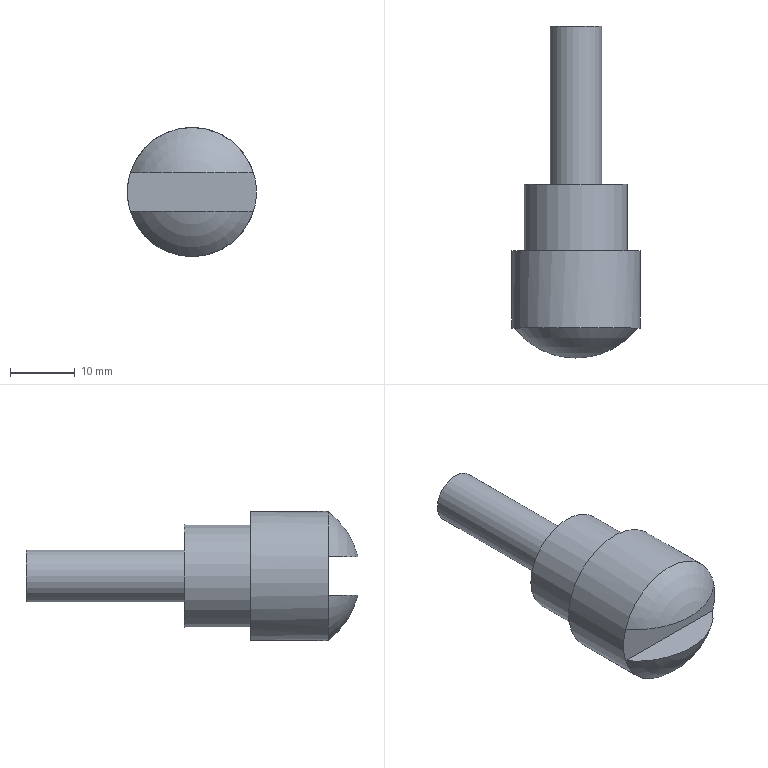Component | NX | 5_STUD | 1 solid | 11 faces | box 20 x 51.43 x 20 mm | volume 7520 mm3 | plane 6 | cylinder 3 | sphere 2 | commonest cylinder face diameters 20 x1 16 x1 8 x1
STEP:
#1=CARTESIAN_POINT('',(0.,0.,0.));
#2=DIRECTION('',(0.,0.,1.));
#3=DIRECTION('',(1.,0.,0.));
#4=AXIS2_PLACEMENT_3D('',#1,#2,#3);
#5=CARTESIAN_POINT('',(11.56,-8.37,11.672));
#6=VERTEX_POINT('',#5);
#7=CARTESIAN_POINT('',(-7.519,-8.37,11.672));
#8=VERTEX_POINT('',#7);
#9=CARTESIAN_POINT('',(2.02,-8.37,14.672));
#10=DIRECTION('',(0.,1.,0.));
#11=DIRECTION('',(1.,0.,0.));
#12=AXIS2_PLACEMENT_3D('',#9,#10,#11);
#13=CIRCLE('',#12,10.);
#14=CARTESIAN_POINT('',(2.02,-0.8696,14.672));
#15=DIRECTION('',(0.,1.,0.));
#16=DIRECTION('',(0.,0.,1.));
#17=AXIS2_PLACEMENT_3D('',#14,#15,#16);
#18=SPHERICAL_SURFACE('',#17,12.5);
#19=CARTESIAN_POINT('',(1.571,-0.6435));
#20=DIRECTION('',(1.,0.));
#21=VECTOR('',#20,1.);
#22=LINE('',#19,#21);
#23=(GEOMETRIC_REPRESENTATION_CONTEXT(2)PARAMETRIC_REPRESENTATION_CONTEXT()REPRESENTATION_CONTEXT('',''));
#24=DEFINITIONAL_REPRESENTATION('',(#22),#23);
#25=PCURVE('',#18,#24);
#26=CARTESIAN_POINT('',(2.02,-14.37,14.672));
#27=DIRECTION('',(0.,1.,0.));
#28=DIRECTION('',(1.,0.,0.));
#29=AXIS2_PLACEMENT_3D('',#26,#27,#28);
#30=CYLINDRICAL_SURFACE('',#29,10.);
#31=CARTESIAN_POINT('',(0.,6.));
#32=DIRECTION('',(1.,0.));
#33=VECTOR('',#32,1.);
#34=LINE('',#31,#33);
#35=(GEOMETRIC_REPRESENTATION_CONTEXT(2)PARAMETRIC_REPRESENTATION_CONTEXT()REPRESENTATION_CONTEXT('',''));
#36=DEFINITIONAL_REPRESENTATION('',(#34),#35);
#37=PCURVE('',#30,#36);
#38=SURFACE_CURVE('',#13,(#25,#37),.PCURVE_S1.);
#39=EDGE_CURVE('',#6,#8,#38,.T.);
#40=ORIENTED_EDGE('',*,*,#39,.F.);
#41=CARTESIAN_POINT('',(2.02,-0.8696,11.672));
#42=DIRECTION('',(0.,0.,-1.));
#43=DIRECTION('',(1.,0.,0.));
#44=AXIS2_PLACEMENT_3D('',#41,#42,#43);
#45=CIRCLE('',#44,12.135);
#46=CARTESIAN_POINT('',(1.875,-0.6435));
#47=CARTESIAN_POINT('',(1.882,-0.6696));
#48=CARTESIAN_POINT('',(1.895,-0.7218));
#49=CARTESIAN_POINT('',(1.921,-0.7994));
#50=CARTESIAN_POINT('',(1.954,-0.8762));
#51=CARTESIAN_POINT('',(1.995,-0.9519));
#52=CARTESIAN_POINT('',(2.049,-1.026));
#53=CARTESIAN_POINT('',(2.12,-1.098));
#54=CARTESIAN_POINT('',(2.218,-1.166));
#55=CARTESIAN_POINT('',(2.353,-1.228));
#56=CARTESIAN_POINT('',(2.544,-1.281));
#57=CARTESIAN_POINT('',(2.81,-1.319));
#58=CARTESIAN_POINT('',(3.142,-1.333));
#59=CARTESIAN_POINT('',(3.473,-1.319));
#60=CARTESIAN_POINT('',(3.739,-1.281));
#61=CARTESIAN_POINT('',(3.93,-1.228));
#62=CARTESIAN_POINT('',(4.065,-1.166));
#63=CARTESIAN_POINT('',(4.163,-1.098));
#64=CARTESIAN_POINT('',(4.234,-1.026));
#65=CARTESIAN_POINT('',(4.288,-0.9519));
#66=CARTESIAN_POINT('',(4.33,-0.8762));
#67=CARTESIAN_POINT('',(4.362,-0.7994));
#68=CARTESIAN_POINT('',(4.388,-0.7218));
#69=CARTESIAN_POINT('',(4.401,-0.6696));
#70=CARTESIAN_POINT('',(4.408,-0.6435));
#71=B_SPLINE_CURVE_WITH_KNOTS('',3,(#46,#47,#48,#49,#50,#51,#52,#53,#54,#55,#56,#57,#58,#59,#60,#61,#62,#63,#64,#65,#66,#67,#68,#69,#70),.UNSPECIFIED.,.F.,.F.,(4,1,1,1,1,1,1,1,1,1,1,1,1,1,1,1,1,1,1,1,1,1,4),(0.6663,0.7485,0.8307,0.913,0.9952,1.077,1.16,1.242,1.324,1.406,1.489,1.571,1.653,1.735,1.817,1.9,1.982,2.064,2.146,2.229,2.311,2.393,2.475),.QUASI_UNIFORM_KNOTS.);
#72=(GEOMETRIC_REPRESENTATION_CONTEXT(2)PARAMETRIC_REPRESENTATION_CONTEXT()REPRESENTATION_CONTEXT('',''));
#73=DEFINITIONAL_REPRESENTATION('',(#71),#72);
#74=PCURVE('',#18,#73);
#75=CARTESIAN_POINT('',(12.02,-8.37,11.672));
#76=DIRECTION('',(-0.,0.,1.));
#77=DIRECTION('',(1.,0.,0.));
#78=AXIS2_PLACEMENT_3D('',#75,#76,#77);
#79=PLANE('',#78);
#80=CARTESIAN_POINT('',(2.135,7.5));
#81=CARTESIAN_POINT('',(2.135,-13.518));
#82=CARTESIAN_POINT('',(-16.067,-3.009));
#83=CARTESIAN_POINT('',(-34.269,7.5));
#84=CARTESIAN_POINT('',(-16.067,18.009));
#85=CARTESIAN_POINT('',(2.135,28.518));
#86=CARTESIAN_POINT('',(2.135,7.5));
#87=(BOUNDED_CURVE()B_SPLINE_CURVE(2,(#80,#81,#82,#83,#84,#85,#86),.UNSPECIFIED.,.T.,.F.)B_SPLINE_CURVE_WITH_KNOTS((1,2,2,2,2,1),(-2.094,0.,2.094,4.189,6.283,8.378),.UNSPECIFIED.)CURVE()GEOMETRIC_REPRESENTATION_ITEM()RATIONAL_B_SPLINE_CURVE((1.,0.5,1.,0.5,1.,0.5,1.))REPRESENTATION_ITEM(''));
#88=(GEOMETRIC_REPRESENTATION_CONTEXT(2)PARAMETRIC_REPRESENTATION_CONTEXT()REPRESENTATION_CONTEXT('',''));
#89=DEFINITIONAL_REPRESENTATION('',(#87),#88);
#90=PCURVE('',#79,#89);
#91=SURFACE_CURVE('',#45,(#74,#90),.PCURVE_S1.);
#92=EDGE_CURVE('',#6,#8,#91,.T.);
#93=ORIENTED_EDGE('',*,*,#92,.T.);
#94=EDGE_LOOP('',(#40,#93));
#95=FACE_BOUND('',#94,.T.);
#96=ADVANCED_FACE('',(#95),#18,.T.);
#97=CARTESIAN_POINT('',(12.02,3.63,14.672));
#98=VERTEX_POINT('',#97);
#99=CARTESIAN_POINT('',(2.02,3.63,14.672));
#100=DIRECTION('',(0.,-1.,0.));
#101=DIRECTION('',(1.,0.,0.));
#102=AXIS2_PLACEMENT_3D('',#99,#100,#101);
#103=CIRCLE('',#102,10.);
#104=CARTESIAN_POINT('',(6.283,18.));
#105=DIRECTION('',(-1.,0.));
#106=VECTOR('',#105,1.);
#107=LINE('',#104,#106);
#108=(GEOMETRIC_REPRESENTATION_CONTEXT(2)PARAMETRIC_REPRESENTATION_CONTEXT()REPRESENTATION_CONTEXT('',''));
#109=DEFINITIONAL_REPRESENTATION('',(#107),#108);
#110=PCURVE('',#30,#109);
#111=CARTESIAN_POINT('',(2.02,3.63,14.672));
#112=DIRECTION('',(0.,1.,0.));
#113=DIRECTION('',(1.,0.,0.));
#114=AXIS2_PLACEMENT_3D('',#111,#112,#113);
#115=PLANE('',#114);
#116=CARTESIAN_POINT('',(10.,0.));
#117=CARTESIAN_POINT('',(10.,-17.321));
#118=CARTESIAN_POINT('',(-5.,-8.66));
#119=CARTESIAN_POINT('',(-20.,-0.));
#120=CARTESIAN_POINT('',(-5.,8.66));
#121=CARTESIAN_POINT('',(10.,17.321));
#122=CARTESIAN_POINT('',(10.,0.));
#123=(BOUNDED_CURVE()B_SPLINE_CURVE(2,(#116,#117,#118,#119,#120,#121,#122),.UNSPECIFIED.,.T.,.F.)B_SPLINE_CURVE_WITH_KNOTS((1,2,2,2,2,1),(-2.094,0.,2.094,4.189,6.283,8.378),.UNSPECIFIED.)CURVE()GEOMETRIC_REPRESENTATION_ITEM()RATIONAL_B_SPLINE_CURVE((1.,0.5,1.,0.5,1.,0.5,1.))REPRESENTATION_ITEM(''));
#124=(GEOMETRIC_REPRESENTATION_CONTEXT(2)PARAMETRIC_REPRESENTATION_CONTEXT()REPRESENTATION_CONTEXT('',''));
#125=DEFINITIONAL_REPRESENTATION('',(#123),#124);
#126=PCURVE('',#115,#125);
#127=SURFACE_CURVE('',#103,(#110,#126),.PCURVE_S1.);
#128=EDGE_CURVE('',#98,#98,#127,.T.);
#129=ORIENTED_EDGE('',*,*,#128,.T.);
#130=CARTESIAN_POINT('',(12.02,-8.37,14.672));
#131=VERTEX_POINT('',#130);
#132=CARTESIAN_POINT('',(12.02,-8.37,14.672));
#133=CARTESIAN_POINT('',(12.02,3.63,14.672));
#134=B_SPLINE_CURVE_WITH_KNOTS('',1,(#132,#133),.UNSPECIFIED.,.F.,.F.,(2,2),(6.,18.),.PIECEWISE_BEZIER_KNOTS.);
#135=CARTESIAN_POINT('',(0.,0.));
#136=DIRECTION('',(0.,1.));
#137=VECTOR('',#136,1.);
#138=LINE('',#135,#137);
#139=(GEOMETRIC_REPRESENTATION_CONTEXT(2)PARAMETRIC_REPRESENTATION_CONTEXT()REPRESENTATION_CONTEXT('',''));
#140=DEFINITIONAL_REPRESENTATION('',(#138),#139);
#141=PCURVE('',#30,#140);
#142=CARTESIAN_POINT('',(6.283,0.));
#143=DIRECTION('',(0.,1.));
#144=VECTOR('',#143,1.);
#145=LINE('',#142,#144);
#146=(GEOMETRIC_REPRESENTATION_CONTEXT(2)PARAMETRIC_REPRESENTATION_CONTEXT()REPRESENTATION_CONTEXT('',''));
#147=DEFINITIONAL_REPRESENTATION('',(#145),#146);
#148=PCURVE('',#30,#147);
#149=SEAM_CURVE('',#134,(#141,#148),.PCURVE_S1.);
#150=EDGE_CURVE('',#131,#98,#149,.T.);
#151=ORIENTED_EDGE('',*,*,#150,.F.);
#152=CARTESIAN_POINT('',(2.02,-8.37,14.672));
#153=DIRECTION('',(0.,1.,0.));
#154=DIRECTION('',(1.,0.,0.));
#155=AXIS2_PLACEMENT_3D('',#152,#153,#154);
#156=CIRCLE('',#155,10.);
#157=CARTESIAN_POINT('',(-6.283,6.));
#158=DIRECTION('',(1.,0.));
#159=VECTOR('',#158,1.);
#160=LINE('',#157,#159);
#161=(GEOMETRIC_REPRESENTATION_CONTEXT(2)PARAMETRIC_REPRESENTATION_CONTEXT()REPRESENTATION_CONTEXT('',''));
#162=DEFINITIONAL_REPRESENTATION('',(#160),#161);
#163=PCURVE('',#30,#162);
#164=CARTESIAN_POINT('',(12.02,-8.37,14.672));
#165=DIRECTION('',(0.,1.,0.));
#166=DIRECTION('',(-1.,0.,-0.));
#167=AXIS2_PLACEMENT_3D('',#164,#165,#166);
#168=PLANE('',#167);
#169=CARTESIAN_POINT('',(10.,0.));
#170=DIRECTION('',(-1.,-0.));
#171=AXIS2_PLACEMENT_2D('',#169,#170);
#172=CIRCLE('',#171,10.);
#173=(GEOMETRIC_REPRESENTATION_CONTEXT(2)PARAMETRIC_REPRESENTATION_CONTEXT()REPRESENTATION_CONTEXT('',''));
#174=DEFINITIONAL_REPRESENTATION('',(#172),#173);
#175=PCURVE('',#168,#174);
#176=SURFACE_CURVE('',#156,(#163,#175),.PCURVE_S1.);
#177=EDGE_CURVE('',#131,#6,#176,.T.);
#178=ORIENTED_EDGE('',*,*,#177,.T.);
#179=ORIENTED_EDGE('',*,*,#39,.T.);
#180=CARTESIAN_POINT('',(-7.519,-8.37,17.672));
#181=VERTEX_POINT('',#180);
#182=CARTESIAN_POINT('',(2.02,-8.37,14.672));
#183=DIRECTION('',(0.,1.,0.));
#184=DIRECTION('',(1.,0.,0.));
#185=AXIS2_PLACEMENT_3D('',#182,#183,#184);
#186=CIRCLE('',#185,10.);
#187=CARTESIAN_POINT('',(0.,6.));
#188=DIRECTION('',(1.,0.));
#189=VECTOR('',#188,1.);
#190=LINE('',#187,#189);
#191=(GEOMETRIC_REPRESENTATION_CONTEXT(2)PARAMETRIC_REPRESENTATION_CONTEXT()REPRESENTATION_CONTEXT('',''));
#192=DEFINITIONAL_REPRESENTATION('',(#190),#191);
#193=PCURVE('',#30,#192);
#194=CARTESIAN_POINT('',(10.,0.));
#195=DIRECTION('',(-1.,-0.));
#196=AXIS2_PLACEMENT_2D('',#194,#195);
#197=CIRCLE('',#196,10.);
#198=(GEOMETRIC_REPRESENTATION_CONTEXT(2)PARAMETRIC_REPRESENTATION_CONTEXT()REPRESENTATION_CONTEXT('',''));
#199=DEFINITIONAL_REPRESENTATION('',(#197),#198);
#200=PCURVE('',#168,#199);
#201=SURFACE_CURVE('',#186,(#193,#200),.PCURVE_S1.);
#202=EDGE_CURVE('',#8,#181,#201,.T.);
#203=ORIENTED_EDGE('',*,*,#202,.T.);
#204=CARTESIAN_POINT('',(11.56,-8.37,17.672));
#205=VERTEX_POINT('',#204);
#206=CARTESIAN_POINT('',(2.02,-8.37,14.672));
#207=DIRECTION('',(0.,1.,0.));
#208=DIRECTION('',(1.,0.,0.));
#209=AXIS2_PLACEMENT_3D('',#206,#207,#208);
#210=CIRCLE('',#209,10.);
#211=CARTESIAN_POINT('',(0.,6.));
#212=DIRECTION('',(1.,0.));
#213=VECTOR('',#212,1.);
#214=LINE('',#211,#213);
#215=(GEOMETRIC_REPRESENTATION_CONTEXT(2)PARAMETRIC_REPRESENTATION_CONTEXT()REPRESENTATION_CONTEXT('',''));
#216=DEFINITIONAL_REPRESENTATION('',(#214),#215);
#217=PCURVE('',#30,#216);
#218=CARTESIAN_POINT('',(2.02,-0.8696,14.672));
#219=DIRECTION('',(0.,1.,0.));
#220=DIRECTION('',(0.,0.,1.));
#221=AXIS2_PLACEMENT_3D('',#218,#219,#220);
#222=SPHERICAL_SURFACE('',#221,12.5);
#223=CARTESIAN_POINT('',(-1.266,-0.6435));
#224=CARTESIAN_POINT('',(-1.228,-0.6435));
#225=CARTESIAN_POINT('',(-1.151,-0.6435));
#226=CARTESIAN_POINT('',(-1.036,-0.6435));
#227=CARTESIAN_POINT('',(-0.9208,-0.6435));
#228=CARTESIAN_POINT('',(-0.8057,-0.6435));
#229=CARTESIAN_POINT('',(-0.6906,-0.6435));
#230=CARTESIAN_POINT('',(-0.5755,-0.6435));
#231=CARTESIAN_POINT('',(-0.4604,-0.6435));
#232=CARTESIAN_POINT('',(-0.3453,-0.6435));
#233=CARTESIAN_POINT('',(-0.2302,-0.6435));
#234=CARTESIAN_POINT('',(-0.1151,-0.6435));
#235=CARTESIAN_POINT('',(0.,-0.6435));
#236=CARTESIAN_POINT('',(0.1151,-0.6435));
#237=CARTESIAN_POINT('',(0.2302,-0.6435));
#238=CARTESIAN_POINT('',(0.3453,-0.6435));
#239=CARTESIAN_POINT('',(0.4604,-0.6435));
#240=CARTESIAN_POINT('',(0.5755,-0.6435));
#241=CARTESIAN_POINT('',(0.6906,-0.6435));
#242=CARTESIAN_POINT('',(0.8057,-0.6435));
#243=CARTESIAN_POINT('',(0.9208,-0.6435));
#244=CARTESIAN_POINT('',(1.036,-0.6435));
#245=CARTESIAN_POINT('',(1.151,-0.6435));
#246=CARTESIAN_POINT('',(1.228,-0.6435));
#247=CARTESIAN_POINT('',(1.266,-0.6435));
#248=B_SPLINE_CURVE_WITH_KNOTS('',3,(#223,#224,#225,#226,#227,#228,#229,#230,#231,#232,#233,#234,#235,#236,#237,#238,#239,#240,#241,#242,#243,#244,#245,#246,#247),.UNSPECIFIED.,.F.,.F.,(4,1,1,1,1,1,1,1,1,1,1,1,1,1,1,1,1,1,1,1,1,1,4),(3.446,3.561,3.676,3.792,3.907,4.022,4.137,4.252,4.367,4.482,4.597,4.712,4.827,4.943,5.058,5.173,5.288,5.403,5.518,5.633,5.748,5.863,5.978),.QUASI_UNIFORM_KNOTS.);
#249=(GEOMETRIC_REPRESENTATION_CONTEXT(2)PARAMETRIC_REPRESENTATION_CONTEXT()REPRESENTATION_CONTEXT('',''));
#250=DEFINITIONAL_REPRESENTATION('',(#248),#249);
#251=PCURVE('',#222,#250);
#252=SURFACE_CURVE('',#210,(#217,#251),.PCURVE_S1.);
#253=EDGE_CURVE('',#181,#205,#252,.T.);
#254=ORIENTED_EDGE('',*,*,#253,.T.);
#255=CARTESIAN_POINT('',(2.02,-8.37,14.672));
#256=DIRECTION('',(0.,1.,0.));
#257=DIRECTION('',(1.,0.,0.));
#258=AXIS2_PLACEMENT_3D('',#255,#256,#257);
#259=CIRCLE('',#258,10.);
#260=CARTESIAN_POINT('',(0.,6.));
#261=DIRECTION('',(1.,0.));
#262=VECTOR('',#261,1.);
#263=LINE('',#260,#262);
#264=(GEOMETRIC_REPRESENTATION_CONTEXT(2)PARAMETRIC_REPRESENTATION_CONTEXT()REPRESENTATION_CONTEXT('',''));
#265=DEFINITIONAL_REPRESENTATION('',(#263),#264);
#266=PCURVE('',#30,#265);
#267=CARTESIAN_POINT('',(10.,0.));
#268=DIRECTION('',(-1.,-0.));
#269=AXIS2_PLACEMENT_2D('',#267,#268);
#270=CIRCLE('',#269,10.);
#271=(GEOMETRIC_REPRESENTATION_CONTEXT(2)PARAMETRIC_REPRESENTATION_CONTEXT()REPRESENTATION_CONTEXT('',''));
#272=DEFINITIONAL_REPRESENTATION('',(#270),#271);
#273=PCURVE('',#168,#272);
#274=SURFACE_CURVE('',#259,(#266,#273),.PCURVE_S1.);
#275=EDGE_CURVE('',#205,#131,#274,.T.);
#276=ORIENTED_EDGE('',*,*,#275,.T.);
#277=ORIENTED_EDGE('',*,*,#150,.T.);
#278=EDGE_LOOP('',(#129,#151,#178,#179,#203,#254,#276,#277));
#279=FACE_BOUND('',#278,.T.);
#280=ADVANCED_FACE('',(#279),#30,.T.);
#281=CARTESIAN_POINT('',(10.02,3.63,14.672));
#282=VERTEX_POINT('',#281);
#283=CARTESIAN_POINT('',(2.02,3.63,14.672));
#284=DIRECTION('',(0.,1.,0.));
#285=DIRECTION('',(1.,0.,0.));
#286=AXIS2_PLACEMENT_3D('',#283,#284,#285);
#287=CIRCLE('',#286,8.);
#288=CARTESIAN_POINT('',(0.,0.));
#289=DIRECTION('',(1.,0.));
#290=AXIS2_PLACEMENT_2D('',#288,#289);
#291=CIRCLE('',#290,8.);
#292=(GEOMETRIC_REPRESENTATION_CONTEXT(2)PARAMETRIC_REPRESENTATION_CONTEXT()REPRESENTATION_CONTEXT('',''));
#293=DEFINITIONAL_REPRESENTATION('',(#291),#292);
#294=PCURVE('',#115,#293);
#295=CARTESIAN_POINT('',(2.02,3.63,14.672));
#296=DIRECTION('',(0.,1.,0.));
#297=DIRECTION('',(1.,0.,0.));
#298=AXIS2_PLACEMENT_3D('',#295,#296,#297);
#299=CYLINDRICAL_SURFACE('',#298,8.);
#300=CARTESIAN_POINT('',(0.,0.));
#301=DIRECTION('',(1.,0.));
#302=VECTOR('',#301,1.);
#303=LINE('',#300,#302);
#304=(GEOMETRIC_REPRESENTATION_CONTEXT(2)PARAMETRIC_REPRESENTATION_CONTEXT()REPRESENTATION_CONTEXT('',''));
#305=DEFINITIONAL_REPRESENTATION('',(#303),#304);
#306=PCURVE('',#299,#305);
#307=SURFACE_CURVE('',#287,(#294,#306),.PCURVE_S1.);
#308=EDGE_CURVE('',#282,#282,#307,.T.);
#309=ORIENTED_EDGE('',*,*,#308,.F.);
#310=EDGE_LOOP('',(#309));
#311=FACE_BOUND('',#310,.T.);
#312=ORIENTED_EDGE('',*,*,#128,.F.);
#313=EDGE_LOOP('',(#312));
#314=FACE_BOUND('',#313,.T.);
#315=ADVANCED_FACE('',(#311,#314),#115,.T.);
#316=CARTESIAN_POINT('',(6.02,13.93,14.672));
#317=VERTEX_POINT('',#316);
#318=CARTESIAN_POINT('',(2.02,13.93,14.672));
#319=DIRECTION('',(0.,1.,0.));
#320=DIRECTION('',(1.,0.,0.));
#321=AXIS2_PLACEMENT_3D('',#318,#319,#320);
#322=CIRCLE('',#321,4.);
#323=CARTESIAN_POINT('',(2.02,13.93,14.672));
#324=DIRECTION('',(0.,1.,0.));
#325=DIRECTION('',(1.,0.,0.));
#326=AXIS2_PLACEMENT_3D('',#323,#324,#325);
#327=PLANE('',#326);
#328=CARTESIAN_POINT('',(0.,0.));
#329=DIRECTION('',(1.,0.));
#330=AXIS2_PLACEMENT_2D('',#328,#329);
#331=CIRCLE('',#330,4.);
#332=(GEOMETRIC_REPRESENTATION_CONTEXT(2)PARAMETRIC_REPRESENTATION_CONTEXT()REPRESENTATION_CONTEXT('',''));
#333=DEFINITIONAL_REPRESENTATION('',(#331),#332);
#334=PCURVE('',#327,#333);
#335=CARTESIAN_POINT('',(2.02,13.93,14.672));
#336=DIRECTION('',(0.,1.,0.));
#337=DIRECTION('',(1.,0.,0.));
#338=AXIS2_PLACEMENT_3D('',#335,#336,#337);
#339=CYLINDRICAL_SURFACE('',#338,4.);
#340=CARTESIAN_POINT('',(0.,0.));
#341=DIRECTION('',(1.,0.));
#342=VECTOR('',#341,1.);
#343=LINE('',#340,#342);
#344=(GEOMETRIC_REPRESENTATION_CONTEXT(2)PARAMETRIC_REPRESENTATION_CONTEXT()REPRESENTATION_CONTEXT('',''));
#345=DEFINITIONAL_REPRESENTATION('',(#343),#344);
#346=PCURVE('',#339,#345);
#347=SURFACE_CURVE('',#322,(#334,#346),.PCURVE_S1.);
#348=EDGE_CURVE('',#317,#317,#347,.T.);
#349=ORIENTED_EDGE('',*,*,#348,.F.);
#350=EDGE_LOOP('',(#349));
#351=FACE_BOUND('',#350,.T.);
#352=CARTESIAN_POINT('',(10.02,13.93,14.672));
#353=VERTEX_POINT('',#352);
#354=CARTESIAN_POINT('',(2.02,13.93,14.672));
#355=DIRECTION('',(0.,-1.,0.));
#356=DIRECTION('',(1.,0.,0.));
#357=AXIS2_PLACEMENT_3D('',#354,#355,#356);
#358=CIRCLE('',#357,8.);
#359=CARTESIAN_POINT('',(8.,0.));
#360=CARTESIAN_POINT('',(8.,-13.856));
#361=CARTESIAN_POINT('',(-4.,-6.928));
#362=CARTESIAN_POINT('',(-16.,-0.));
#363=CARTESIAN_POINT('',(-4.,6.928));
#364=CARTESIAN_POINT('',(8.,13.856));
#365=CARTESIAN_POINT('',(8.,0.));
#366=(BOUNDED_CURVE()B_SPLINE_CURVE(2,(#359,#360,#361,#362,#363,#364,#365),.UNSPECIFIED.,.T.,.F.)B_SPLINE_CURVE_WITH_KNOTS((1,2,2,2,2,1),(-2.094,0.,2.094,4.189,6.283,8.378),.UNSPECIFIED.)CURVE()GEOMETRIC_REPRESENTATION_ITEM()RATIONAL_B_SPLINE_CURVE((1.,0.5,1.,0.5,1.,0.5,1.))REPRESENTATION_ITEM(''));
#367=(GEOMETRIC_REPRESENTATION_CONTEXT(2)PARAMETRIC_REPRESENTATION_CONTEXT()REPRESENTATION_CONTEXT('',''));
#368=DEFINITIONAL_REPRESENTATION('',(#366),#367);
#369=PCURVE('',#327,#368);
#370=CARTESIAN_POINT('',(6.283,10.3));
#371=DIRECTION('',(-1.,0.));
#372=VECTOR('',#371,1.);
#373=LINE('',#370,#372);
#374=(GEOMETRIC_REPRESENTATION_CONTEXT(2)PARAMETRIC_REPRESENTATION_CONTEXT()REPRESENTATION_CONTEXT('',''));
#375=DEFINITIONAL_REPRESENTATION('',(#373),#374);
#376=PCURVE('',#299,#375);
#377=SURFACE_CURVE('',#358,(#369,#376),.PCURVE_S1.);
#378=EDGE_CURVE('',#353,#353,#377,.T.);
#379=ORIENTED_EDGE('',*,*,#378,.F.);
#380=EDGE_LOOP('',(#379));
#381=FACE_BOUND('',#380,.T.);
#382=ADVANCED_FACE('',(#351,#381),#327,.T.);
#383=ORIENTED_EDGE('',*,*,#378,.T.);
#384=CARTESIAN_POINT('',(10.02,3.63,14.672));
#385=CARTESIAN_POINT('',(10.02,13.93,14.672));
#386=B_SPLINE_CURVE_WITH_KNOTS('',1,(#384,#385),.UNSPECIFIED.,.F.,.F.,(2,2),(0.,10.3),.PIECEWISE_BEZIER_KNOTS.);
#387=CARTESIAN_POINT('',(0.,0.));
#388=DIRECTION('',(0.,1.));
#389=VECTOR('',#388,1.);
#390=LINE('',#387,#389);
#391=(GEOMETRIC_REPRESENTATION_CONTEXT(2)PARAMETRIC_REPRESENTATION_CONTEXT()REPRESENTATION_CONTEXT('',''));
#392=DEFINITIONAL_REPRESENTATION('',(#390),#391);
#393=PCURVE('',#299,#392);
#394=CARTESIAN_POINT('',(6.283,0.));
#395=DIRECTION('',(0.,1.));
#396=VECTOR('',#395,1.);
#397=LINE('',#394,#396);
#398=(GEOMETRIC_REPRESENTATION_CONTEXT(2)PARAMETRIC_REPRESENTATION_CONTEXT()REPRESENTATION_CONTEXT('',''));
#399=DEFINITIONAL_REPRESENTATION('',(#397),#398);
#400=PCURVE('',#299,#399);
#401=SEAM_CURVE('',#386,(#393,#400),.PCURVE_S1.);
#402=EDGE_CURVE('',#282,#353,#401,.T.);
#403=ORIENTED_EDGE('',*,*,#402,.F.);
#404=ORIENTED_EDGE('',*,*,#308,.T.);
#405=ORIENTED_EDGE('',*,*,#402,.T.);
#406=EDGE_LOOP('',(#383,#403,#404,#405));
#407=FACE_BOUND('',#406,.T.);
#408=ADVANCED_FACE('',(#407),#299,.T.);
#409=CARTESIAN_POINT('',(6.02,38.43,14.672));
#410=VERTEX_POINT('',#409);
#411=CARTESIAN_POINT('',(2.02,38.43,14.672));
#412=DIRECTION('',(0.,-1.,0.));
#413=DIRECTION('',(1.,0.,0.));
#414=AXIS2_PLACEMENT_3D('',#411,#412,#413);
#415=CIRCLE('',#414,4.);
#416=CARTESIAN_POINT('',(2.02,38.43,14.672));
#417=DIRECTION('',(0.,1.,0.));
#418=DIRECTION('',(1.,0.,0.));
#419=AXIS2_PLACEMENT_3D('',#416,#417,#418);
#420=PLANE('',#419);
#421=CARTESIAN_POINT('',(4.,0.));
#422=CARTESIAN_POINT('',(4.,-6.928));
#423=CARTESIAN_POINT('',(-2.,-3.464));
#424=CARTESIAN_POINT('',(-8.,-0.));
#425=CARTESIAN_POINT('',(-2.,3.464));
#426=CARTESIAN_POINT('',(4.,6.928));
#427=CARTESIAN_POINT('',(4.,0.));
#428=(BOUNDED_CURVE()B_SPLINE_CURVE(2,(#421,#422,#423,#424,#425,#426,#427),.UNSPECIFIED.,.T.,.F.)B_SPLINE_CURVE_WITH_KNOTS((1,2,2,2,2,1),(-2.094,0.,2.094,4.189,6.283,8.378),.UNSPECIFIED.)CURVE()GEOMETRIC_REPRESENTATION_ITEM()RATIONAL_B_SPLINE_CURVE((1.,0.5,1.,0.5,1.,0.5,1.))REPRESENTATION_ITEM(''));
#429=(GEOMETRIC_REPRESENTATION_CONTEXT(2)PARAMETRIC_REPRESENTATION_CONTEXT()REPRESENTATION_CONTEXT('',''));
#430=DEFINITIONAL_REPRESENTATION('',(#428),#429);
#431=PCURVE('',#420,#430);
#432=CARTESIAN_POINT('',(6.283,24.5));
#433=DIRECTION('',(-1.,0.));
#434=VECTOR('',#433,1.);
#435=LINE('',#432,#434);
#436=(GEOMETRIC_REPRESENTATION_CONTEXT(2)PARAMETRIC_REPRESENTATION_CONTEXT()REPRESENTATION_CONTEXT('',''));
#437=DEFINITIONAL_REPRESENTATION('',(#435),#436);
#438=PCURVE('',#339,#437);
#439=SURFACE_CURVE('',#415,(#431,#438),.PCURVE_S1.);
#440=EDGE_CURVE('',#410,#410,#439,.T.);
#441=ORIENTED_EDGE('',*,*,#440,.F.);
#442=EDGE_LOOP('',(#441));
#443=FACE_BOUND('',#442,.T.);
#444=ADVANCED_FACE('',(#443),#420,.T.);
#445=ORIENTED_EDGE('',*,*,#440,.T.);
#446=CARTESIAN_POINT('',(6.02,13.93,14.672));
#447=CARTESIAN_POINT('',(6.02,38.43,14.672));
#448=B_SPLINE_CURVE_WITH_KNOTS('',1,(#446,#447),.UNSPECIFIED.,.F.,.F.,(2,2),(0.,24.5),.PIECEWISE_BEZIER_KNOTS.);
#449=CARTESIAN_POINT('',(0.,0.));
#450=DIRECTION('',(0.,1.));
#451=VECTOR('',#450,1.);
#452=LINE('',#449,#451);
#453=(GEOMETRIC_REPRESENTATION_CONTEXT(2)PARAMETRIC_REPRESENTATION_CONTEXT()REPRESENTATION_CONTEXT('',''));
#454=DEFINITIONAL_REPRESENTATION('',(#452),#453);
#455=PCURVE('',#339,#454);
#456=CARTESIAN_POINT('',(6.283,0.));
#457=DIRECTION('',(0.,1.));
#458=VECTOR('',#457,1.);
#459=LINE('',#456,#458);
#460=(GEOMETRIC_REPRESENTATION_CONTEXT(2)PARAMETRIC_REPRESENTATION_CONTEXT()REPRESENTATION_CONTEXT('',''));
#461=DEFINITIONAL_REPRESENTATION('',(#459),#460);
#462=PCURVE('',#339,#461);
#463=SEAM_CURVE('',#448,(#455,#462),.PCURVE_S1.);
#464=EDGE_CURVE('',#317,#410,#463,.T.);
#465=ORIENTED_EDGE('',*,*,#464,.F.);
#466=ORIENTED_EDGE('',*,*,#348,.T.);
#467=ORIENTED_EDGE('',*,*,#464,.T.);
#468=EDGE_LOOP('',(#445,#465,#466,#467));
#469=FACE_BOUND('',#468,.T.);
#470=ADVANCED_FACE('',(#469),#339,.T.);
#471=CARTESIAN_POINT('',(2.02,-0.8696,17.672));
#472=DIRECTION('',(0.,0.,-1.));
#473=DIRECTION('',(1.,0.,0.));
#474=AXIS2_PLACEMENT_3D('',#471,#472,#473);
#475=CIRCLE('',#474,12.135);
#476=CARTESIAN_POINT('',(1.266,-0.6435));
#477=CARTESIAN_POINT('',(1.26,-0.6696));
#478=CARTESIAN_POINT('',(1.246,-0.7218));
#479=CARTESIAN_POINT('',(1.221,-0.7994));
#480=CARTESIAN_POINT('',(1.188,-0.8762));
#481=CARTESIAN_POINT('',(1.147,-0.9519));
#482=CARTESIAN_POINT('',(1.093,-1.026));
#483=CARTESIAN_POINT('',(1.021,-1.098));
#484=CARTESIAN_POINT('',(0.9239,-1.166));
#485=CARTESIAN_POINT('',(0.7885,-1.228));
#486=CARTESIAN_POINT('',(0.5973,-1.281));
#487=CARTESIAN_POINT('',(0.3318,-1.319));
#488=CARTESIAN_POINT('',(0.,-1.333));
#489=CARTESIAN_POINT('',(-0.3318,-1.319));
#490=CARTESIAN_POINT('',(-0.5973,-1.281));
#491=CARTESIAN_POINT('',(-0.7885,-1.228));
#492=CARTESIAN_POINT('',(-0.9239,-1.166));
#493=CARTESIAN_POINT('',(-1.021,-1.098));
#494=CARTESIAN_POINT('',(-1.093,-1.026));
#495=CARTESIAN_POINT('',(-1.147,-0.9519));
#496=CARTESIAN_POINT('',(-1.188,-0.8762));
#497=CARTESIAN_POINT('',(-1.221,-0.7994));
#498=CARTESIAN_POINT('',(-1.246,-0.7218));
#499=CARTESIAN_POINT('',(-1.26,-0.6696));
#500=CARTESIAN_POINT('',(-1.266,-0.6435));
#501=B_SPLINE_CURVE_WITH_KNOTS('',3,(#476,#477,#478,#479,#480,#481,#482,#483,#484,#485,#486,#487,#488,#489,#490,#491,#492,#493,#494,#495,#496,#497,#498,#499,#500),.UNSPECIFIED.,.F.,.F.,(4,1,1,1,1,1,1,1,1,1,1,1,1,1,1,1,1,1,1,1,1,1,4),(0.6663,0.7485,0.8307,0.913,0.9952,1.077,1.16,1.242,1.324,1.406,1.489,1.571,1.653,1.735,1.817,1.9,1.982,2.064,2.146,2.229,2.311,2.393,2.475),.QUASI_UNIFORM_KNOTS.);
#502=(GEOMETRIC_REPRESENTATION_CONTEXT(2)PARAMETRIC_REPRESENTATION_CONTEXT()REPRESENTATION_CONTEXT('',''));
#503=DEFINITIONAL_REPRESENTATION('',(#501),#502);
#504=PCURVE('',#222,#503);
#505=CARTESIAN_POINT('',(12.02,-8.37,17.672));
#506=DIRECTION('',(-0.,0.,1.));
#507=DIRECTION('',(1.,0.,0.));
#508=AXIS2_PLACEMENT_3D('',#505,#506,#507);
#509=PLANE('',#508);
#510=CARTESIAN_POINT('',(2.135,7.5));
#511=CARTESIAN_POINT('',(2.135,-13.518));
#512=CARTESIAN_POINT('',(-16.067,-3.009));
#513=CARTESIAN_POINT('',(-34.269,7.5));
#514=CARTESIAN_POINT('',(-16.067,18.009));
#515=CARTESIAN_POINT('',(2.135,28.518));
#516=CARTESIAN_POINT('',(2.135,7.5));
#517=(BOUNDED_CURVE()B_SPLINE_CURVE(2,(#510,#511,#512,#513,#514,#515,#516),.UNSPECIFIED.,.T.,.F.)B_SPLINE_CURVE_WITH_KNOTS((1,2,2,2,2,1),(-2.094,0.,2.094,4.189,6.283,8.378),.UNSPECIFIED.)CURVE()GEOMETRIC_REPRESENTATION_ITEM()RATIONAL_B_SPLINE_CURVE((1.,0.5,1.,0.5,1.,0.5,1.))REPRESENTATION_ITEM(''));
#518=(GEOMETRIC_REPRESENTATION_CONTEXT(2)PARAMETRIC_REPRESENTATION_CONTEXT()REPRESENTATION_CONTEXT('',''));
#519=DEFINITIONAL_REPRESENTATION('',(#517),#518);
#520=PCURVE('',#509,#519);
#521=SURFACE_CURVE('',#475,(#504,#520),.PCURVE_S1.);
#522=EDGE_CURVE('',#205,#181,#521,.T.);
#523=ORIENTED_EDGE('',*,*,#522,.F.);
#524=ORIENTED_EDGE('',*,*,#253,.F.);
#525=EDGE_LOOP('',(#523,#524));
#526=FACE_BOUND('',#525,.T.);
#527=ADVANCED_FACE('',(#526),#222,.T.);
#528=ORIENTED_EDGE('',*,*,#177,.T.);
#529=CARTESIAN_POINT('',(12.02,-8.37,11.672));
#530=DIRECTION('',(1.,0.,0.));
#531=VECTOR('',#530,1.);
#532=LINE('',#529,#531);
#533=CARTESIAN_POINT('',(0.,-3.));
#534=DIRECTION('',(-1.,0.));
#535=VECTOR('',#534,1.);
#536=LINE('',#533,#535);
#537=(GEOMETRIC_REPRESENTATION_CONTEXT(2)PARAMETRIC_REPRESENTATION_CONTEXT()REPRESENTATION_CONTEXT('',''));
#538=DEFINITIONAL_REPRESENTATION('',(#536),#537);
#539=PCURVE('',#168,#538);
#540=CARTESIAN_POINT('',(0.,0.));
#541=DIRECTION('',(1.,0.));
#542=VECTOR('',#541,1.);
#543=LINE('',#540,#542);
#544=(GEOMETRIC_REPRESENTATION_CONTEXT(2)PARAMETRIC_REPRESENTATION_CONTEXT()REPRESENTATION_CONTEXT('',''));
#545=DEFINITIONAL_REPRESENTATION('',(#543),#544);
#546=PCURVE('',#79,#545);
#547=SURFACE_CURVE('',#532,(#539,#546),.PCURVE_S1.);
#548=EDGE_CURVE('',#8,#6,#547,.T.);
#549=ORIENTED_EDGE('',*,*,#548,.F.);
#550=ORIENTED_EDGE('',*,*,#202,.T.);
#551=CARTESIAN_POINT('',(12.02,-8.37,17.672));
#552=DIRECTION('',(1.,0.,0.));
#553=VECTOR('',#552,1.);
#554=LINE('',#551,#553);
#555=CARTESIAN_POINT('',(-0.,3.));
#556=DIRECTION('',(-1.,0.));
#557=VECTOR('',#556,1.);
#558=LINE('',#555,#557);
#559=(GEOMETRIC_REPRESENTATION_CONTEXT(2)PARAMETRIC_REPRESENTATION_CONTEXT()REPRESENTATION_CONTEXT('',''));
#560=DEFINITIONAL_REPRESENTATION('',(#558),#559);
#561=PCURVE('',#168,#560);
#562=CARTESIAN_POINT('',(0.,0.));
#563=DIRECTION('',(1.,0.));
#564=VECTOR('',#563,1.);
#565=LINE('',#562,#564);
#566=(GEOMETRIC_REPRESENTATION_CONTEXT(2)PARAMETRIC_REPRESENTATION_CONTEXT()REPRESENTATION_CONTEXT('',''));
#567=DEFINITIONAL_REPRESENTATION('',(#565),#566);
#568=PCURVE('',#509,#567);
#569=SURFACE_CURVE('',#554,(#561,#568),.PCURVE_S1.);
#570=EDGE_CURVE('',#181,#205,#569,.T.);
#571=ORIENTED_EDGE('',*,*,#570,.T.);
#572=ORIENTED_EDGE('',*,*,#275,.T.);
#573=EDGE_LOOP('',(#528,#549,#550,#571,#572));
#574=FACE_BOUND('',#573,.F.);
#575=ADVANCED_FACE('',(#574),#168,.F.);
#576=ORIENTED_EDGE('',*,*,#522,.T.);
#577=ORIENTED_EDGE('',*,*,#570,.T.);
#578=EDGE_LOOP('',(#576,#577));
#579=FACE_BOUND('',#578,.T.);
#580=ADVANCED_FACE('',(#579),#509,.F.);
#581=ORIENTED_EDGE('',*,*,#548,.F.);
#582=ORIENTED_EDGE('',*,*,#92,.F.);
#583=EDGE_LOOP('',(#581,#582));
#584=FACE_BOUND('',#583,.T.);
#585=ADVANCED_FACE('',(#584),#79,.T.);
#586=CLOSED_SHELL('',(#96,#280,#315,#382,#408,#444,#470,#527,#575,#580,#585));
#587=MANIFOLD_SOLID_BREP('',#586);
#588=(LENGTH_UNIT()NAMED_UNIT(*)SI_UNIT(.MILLI.,.METRE.));
#589=UNCERTAINTY_MEASURE_WITH_UNIT(LENGTH_MEASURE(0.000005),#588,'','');
#590=(NAMED_UNIT(*)PLANE_ANGLE_UNIT()SI_UNIT($,.RADIAN.));
#591=(NAMED_UNIT(*)SI_UNIT($,.STERADIAN.)SOLID_ANGLE_UNIT());
#592=(GEOMETRIC_REPRESENTATION_CONTEXT(3)GLOBAL_UNCERTAINTY_ASSIGNED_CONTEXT((#589))GLOBAL_UNIT_ASSIGNED_CONTEXT((#588,#590,#591))REPRESENTATION_CONTEXT('',''));
#593=ADVANCED_BREP_SHAPE_REPRESENTATION('',(#4,#587),#592);